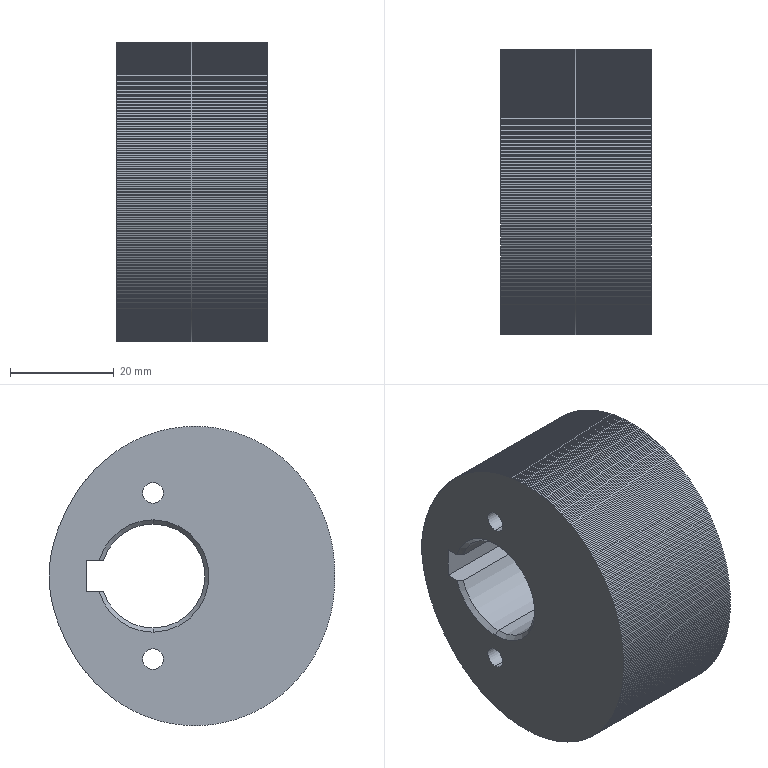Component | SolidWorks | CamGroup4-1_Cam7-1 | 1 solid | 644 faces | volume 61436 mm3 | plane 634 | cylinder 7 | cone 3 | commonest cylinder face diameters 4 x4 20 x3